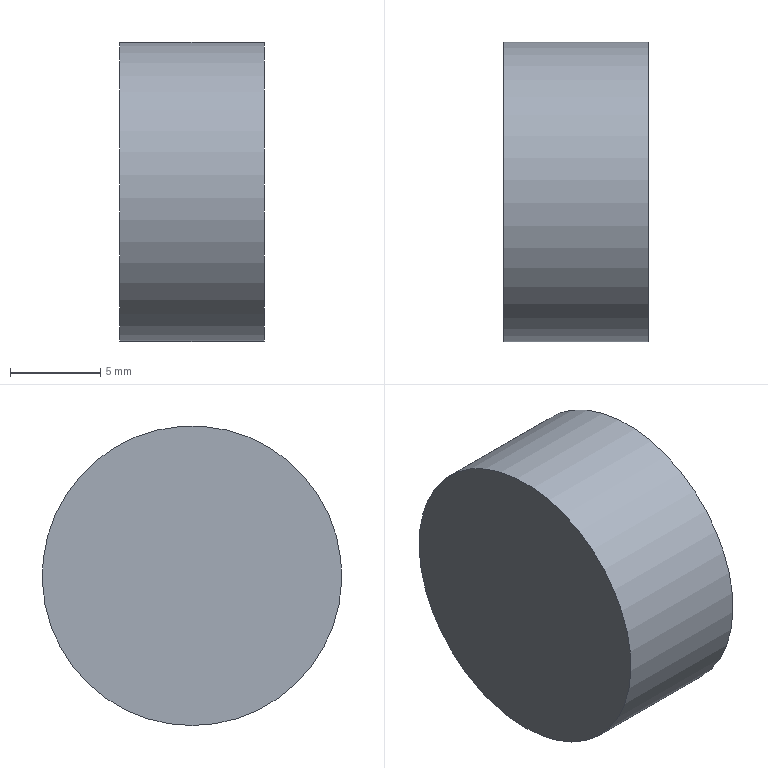Component | NX | VALVE_PORT_FILTER_2 | 1 solid | 3 faces | box 8 x 16.6 x 16.6 mm | volume 1731 mm3 | plane 2 | cylinder 1 | commonest cylinder face diameters 16.6 x1
STEP:
#1=CARTESIAN_POINT('',(0.,0.,0.));
#2=DIRECTION('',(0.,0.,1.));
#3=DIRECTION('',(1.,0.,0.));
#4=AXIS2_PLACEMENT_3D('',#1,#2,#3);
#5=CARTESIAN_POINT('',(6.095,-20.891,-8.3));
#6=VERTEX_POINT('',#5);
#7=CARTESIAN_POINT('',(6.095,-20.891,-0.));
#8=DIRECTION('',(1.,0.,0.));
#9=DIRECTION('',(0.,0.,-1.));
#10=AXIS2_PLACEMENT_3D('',#7,#8,#9);
#11=CIRCLE('',#10,8.3);
#12=CARTESIAN_POINT('',(6.095,-20.891,-0.));
#13=DIRECTION('',(-1.,0.,0.));
#14=DIRECTION('',(0.,0.,1.));
#15=AXIS2_PLACEMENT_3D('',#12,#13,#14);
#16=CYLINDRICAL_SURFACE('',#15,8.3);
#17=CARTESIAN_POINT('',(9.425,0.));
#18=DIRECTION('',(-1.,0.));
#19=VECTOR('',#18,1.);
#20=LINE('',#17,#19);
#21=(GEOMETRIC_REPRESENTATION_CONTEXT(2)PARAMETRIC_REPRESENTATION_CONTEXT()REPRESENTATION_CONTEXT('',''));
#22=DEFINITIONAL_REPRESENTATION('',(#20),#21);
#23=PCURVE('',#16,#22);
#24=CARTESIAN_POINT('',(6.095,-20.891,-0.));
#25=DIRECTION('',(1.,0.,0.));
#26=DIRECTION('',(0.,0.,-1.));
#27=AXIS2_PLACEMENT_3D('',#24,#25,#26);
#28=PLANE('',#27);
#29=CARTESIAN_POINT('',(0.,0.));
#30=DIRECTION('',(1.,0.));
#31=AXIS2_PLACEMENT_2D('',#29,#30);
#32=CIRCLE('',#31,8.3);
#33=(GEOMETRIC_REPRESENTATION_CONTEXT(2)PARAMETRIC_REPRESENTATION_CONTEXT()REPRESENTATION_CONTEXT('',''));
#34=DEFINITIONAL_REPRESENTATION('',(#32),#33);
#35=PCURVE('',#28,#34);
#36=SURFACE_CURVE('',#11,(#23,#35),.PCURVE_S1.);
#37=EDGE_CURVE('',#6,#6,#36,.T.);
#38=ORIENTED_EDGE('',*,*,#37,.F.);
#39=CARTESIAN_POINT('',(-1.905,-20.891,-8.3));
#40=VERTEX_POINT('',#39);
#41=CARTESIAN_POINT('',(6.095,-20.891,-8.3));
#42=CARTESIAN_POINT('',(-1.905,-20.891,-8.3));
#43=B_SPLINE_CURVE_WITH_KNOTS('',1,(#41,#42),.UNSPECIFIED.,.F.,.F.,(2,2),(0.,8.),.PIECEWISE_BEZIER_KNOTS.);
#44=CARTESIAN_POINT('',(9.425,0.));
#45=DIRECTION('',(0.,1.));
#46=VECTOR('',#45,1.);
#47=LINE('',#44,#46);
#48=(GEOMETRIC_REPRESENTATION_CONTEXT(2)PARAMETRIC_REPRESENTATION_CONTEXT()REPRESENTATION_CONTEXT('',''));
#49=DEFINITIONAL_REPRESENTATION('',(#47),#48);
#50=PCURVE('',#16,#49);
#51=CARTESIAN_POINT('',(3.142,0.));
#52=DIRECTION('',(0.,1.));
#53=VECTOR('',#52,1.);
#54=LINE('',#51,#53);
#55=(GEOMETRIC_REPRESENTATION_CONTEXT(2)PARAMETRIC_REPRESENTATION_CONTEXT()REPRESENTATION_CONTEXT('',''));
#56=DEFINITIONAL_REPRESENTATION('',(#54),#55);
#57=PCURVE('',#16,#56);
#58=SEAM_CURVE('',#43,(#50,#57),.PCURVE_S1.);
#59=EDGE_CURVE('',#6,#40,#58,.T.);
#60=ORIENTED_EDGE('',*,*,#59,.T.);
#61=CARTESIAN_POINT('',(-1.905,-20.891,-0.));
#62=DIRECTION('',(1.,0.,0.));
#63=DIRECTION('',(0.,0.,-1.));
#64=AXIS2_PLACEMENT_3D('',#61,#62,#63);
#65=CIRCLE('',#64,8.3);
#66=CARTESIAN_POINT('',(9.425,8.));
#67=DIRECTION('',(-1.,0.));
#68=VECTOR('',#67,1.);
#69=LINE('',#66,#68);
#70=(GEOMETRIC_REPRESENTATION_CONTEXT(2)PARAMETRIC_REPRESENTATION_CONTEXT()REPRESENTATION_CONTEXT('',''));
#71=DEFINITIONAL_REPRESENTATION('',(#69),#70);
#72=PCURVE('',#16,#71);
#73=CARTESIAN_POINT('',(-1.905,-20.891,-0.));
#74=DIRECTION('',(1.,0.,0.));
#75=DIRECTION('',(0.,0.,-1.));
#76=AXIS2_PLACEMENT_3D('',#73,#74,#75);
#77=PLANE('',#76);
#78=CARTESIAN_POINT('',(0.,0.));
#79=DIRECTION('',(1.,0.));
#80=AXIS2_PLACEMENT_2D('',#78,#79);
#81=CIRCLE('',#80,8.3);
#82=(GEOMETRIC_REPRESENTATION_CONTEXT(2)PARAMETRIC_REPRESENTATION_CONTEXT()REPRESENTATION_CONTEXT('',''));
#83=DEFINITIONAL_REPRESENTATION('',(#81),#82);
#84=PCURVE('',#77,#83);
#85=SURFACE_CURVE('',#65,(#72,#84),.PCURVE_S1.);
#86=EDGE_CURVE('',#40,#40,#85,.T.);
#87=ORIENTED_EDGE('',*,*,#86,.T.);
#88=ORIENTED_EDGE('',*,*,#59,.F.);
#89=EDGE_LOOP('',(#38,#60,#87,#88));
#90=FACE_BOUND('',#89,.T.);
#91=ADVANCED_FACE('',(#90),#16,.T.);
#92=ORIENTED_EDGE('',*,*,#37,.T.);
#93=EDGE_LOOP('',(#92));
#94=FACE_BOUND('',#93,.T.);
#95=ADVANCED_FACE('',(#94),#28,.T.);
#96=ORIENTED_EDGE('',*,*,#86,.F.);
#97=EDGE_LOOP('',(#96));
#98=FACE_BOUND('',#97,.T.);
#99=ADVANCED_FACE('',(#98),#77,.F.);
#100=CLOSED_SHELL('',(#91,#95,#99));
#101=MANIFOLD_SOLID_BREP('',#100);
#102=(LENGTH_UNIT()NAMED_UNIT(*)SI_UNIT(.MILLI.,.METRE.));
#103=UNCERTAINTY_MEASURE_WITH_UNIT(LENGTH_MEASURE(0.00001),#102,'','');
#104=(NAMED_UNIT(*)PLANE_ANGLE_UNIT()SI_UNIT($,.RADIAN.));
#105=(NAMED_UNIT(*)SI_UNIT($,.STERADIAN.)SOLID_ANGLE_UNIT());
#106=(GEOMETRIC_REPRESENTATION_CONTEXT(3)GLOBAL_UNCERTAINTY_ASSIGNED_CONTEXT((#103))GLOBAL_UNIT_ASSIGNED_CONTEXT((#102,#104,#105))REPRESENTATION_CONTEXT('',''));
#107=ADVANCED_BREP_SHAPE_REPRESENTATION('',(#4,#101),#106);